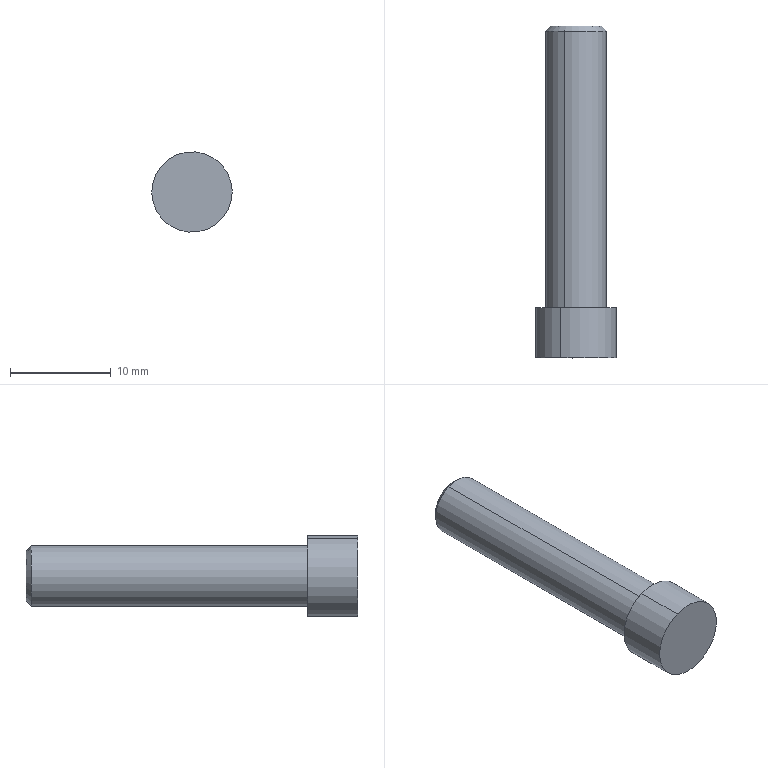Component | SolidWorks | 6x30TPunch-2 | 1 solid | 9 faces | box 8 x 33 x 8 mm | volume 1041 mm3 | cylinder 4 | plane 3 | cone 2 | commonest cylinder face diameters 8 x2 6 x2 | material Cr12
build123d program:
from build123d import *

# Parameters (mm, degrees)
SKETCH1_R           = 3
BOSS_EXTRUDE1_DEPTH = 28
SKETCH2_R           = 4
BOSS_EXTRUDE2_DEPTH = 5
CHAMFER1_SIZE       = 0.5


with BuildPart() as part:
    # Sketch1 → Boss-Extrude1 (new body)
    with BuildSketch(Plane(origin=(0, 0, 0), x_dir=(1, 0, 0), z_dir=(0, 1, 0))):
        with Locations(Location((0, 0, 0), (0, 0, 270))):
            Circle(SKETCH1_R)
    extrude(amount=BOSS_EXTRUDE1_DEPTH)

    # Sketch2 → Boss-Extrude2 (add)
    with BuildSketch(Plane(origin=(0, 28, 0), x_dir=(1, 0, 0), z_dir=(0, 1, 0))):
        with Locations(Location((0, 0, 0), (0, 0, 270))):
            Circle(SKETCH2_R)
    extrude(amount=BOSS_EXTRUDE2_DEPTH)

    # Chamfer1
    chamfer1_edges = [part.edges().sort_by_distance(p)[0] for p in [
        (0, 0, -3),
    ]]
    chamfer(chamfer1_edges, length=CHAMFER1_SIZE)


solid = part.part

# Placed as in the assembly
solid = solid.moved(Location((121.714, -49, 0), (180, 0, 0)))
STEP:
#1=CARTESIAN_POINT('',(4.829,-1.929,-0.09107));
#2=VERTEX_POINT('',#1);
#3=CARTESIAN_POINT('',(4.755,-1.929,0.09107));
#4=VERTEX_POINT('',#3);
#5=CARTESIAN_POINT('',(4.792,-1.929,-0.));
#6=DIRECTION('',(-0.,1.,0.));
#7=DIRECTION('',(-0.3794,0.,0.9252));
#8=AXIS2_PLACEMENT_3D('',#5,#6,#7);
#9=CIRCLE('',#8,0.09843);
#10=EDGE_CURVE('',#2,#4,#9,.T.);
#11=ORIENTED_EDGE('',*,*,#10,.F.);
#12=CARTESIAN_POINT('',(4.837,-1.949,-0.1093));
#13=VERTEX_POINT('',#12);
#14=CARTESIAN_POINT('',(4.837,-1.949,-0.1093));
#15=DIRECTION('',(0.2683,-0.7071,-0.6542));
#16=VECTOR('',#15,39.37);
#17=LINE('',#14,#16);
#18=EDGE_CURVE('',#2,#13,#17,.T.);
#19=ORIENTED_EDGE('',*,*,#18,.T.);
#20=CARTESIAN_POINT('',(4.747,-1.949,0.1093));
#21=VERTEX_POINT('',#20);
#22=CARTESIAN_POINT('',(4.792,-1.949,-0.));
#23=DIRECTION('',(0.,-1.,-0.));
#24=DIRECTION('',(-0.3794,0.,0.9252));
#25=AXIS2_PLACEMENT_3D('',#22,#23,#24);
#26=CIRCLE('',#25,0.1181);
#27=EDGE_CURVE('',#21,#13,#26,.T.);
#28=ORIENTED_EDGE('',*,*,#27,.F.);
#29=CARTESIAN_POINT('',(4.747,-1.949,0.1093));
#30=DIRECTION('',(-0.2683,-0.7071,0.6542));
#31=VECTOR('',#30,39.37);
#32=LINE('',#29,#31);
#33=EDGE_CURVE('',#4,#21,#32,.T.);
#34=ORIENTED_EDGE('',*,*,#33,.F.);
#35=EDGE_LOOP('',(#11,#19,#28,#34));
#36=FACE_OUTER_BOUND('',#35,.T.);
#37=CARTESIAN_POINT('',(4.792,-1.949,-0.));
#38=DIRECTION('',(0.,-1.,-0.));
#39=DIRECTION('',(-0.3794,0.,0.9252));
#40=AXIS2_PLACEMENT_3D('',#37,#38,#39);
#41=CONICAL_SURFACE('',#40,0.1181,0.7854);
#42=ADVANCED_FACE('',(#36),#41,.T.);
#43=CARTESIAN_POINT('',(4.732,-3.228,0.1457));
#44=VERTEX_POINT('',#43);
#45=CARTESIAN_POINT('',(4.852,-3.228,-0.1457));
#46=VERTEX_POINT('',#45);
#47=CARTESIAN_POINT('',(4.792,-3.228,-0.));
#48=DIRECTION('',(0.,-1.,-0.));
#49=DIRECTION('',(-0.3794,0.,0.9252));
#50=AXIS2_PLACEMENT_3D('',#47,#48,#49);
#51=CIRCLE('',#50,0.1575);
#52=EDGE_CURVE('',#44,#46,#51,.T.);
#53=ORIENTED_EDGE('',*,*,#52,.F.);
#54=CARTESIAN_POINT('',(4.732,-3.031,0.1457));
#55=VERTEX_POINT('',#54);
#56=CARTESIAN_POINT('',(4.732,-3.228,0.1457));
#57=DIRECTION('',(-0.,1.,0.));
#58=VECTOR('',#57,39.37);
#59=LINE('',#56,#58);
#60=EDGE_CURVE('',#44,#55,#59,.T.);
#61=ORIENTED_EDGE('',*,*,#60,.T.);
#62=CARTESIAN_POINT('',(4.852,-3.031,-0.1457));
#63=VERTEX_POINT('',#62);
#64=CARTESIAN_POINT('',(4.792,-3.031,-0.));
#65=DIRECTION('',(0.,-1.,-0.));
#66=DIRECTION('',(-0.3794,0.,0.9252));
#67=AXIS2_PLACEMENT_3D('',#64,#65,#66);
#68=CIRCLE('',#67,0.1575);
#69=EDGE_CURVE('',#55,#63,#68,.T.);
#70=ORIENTED_EDGE('',*,*,#69,.T.);
#71=CARTESIAN_POINT('',(4.852,-3.228,-0.1457));
#72=DIRECTION('',(-0.,1.,0.));
#73=VECTOR('',#72,39.37);
#74=LINE('',#71,#73);
#75=EDGE_CURVE('',#46,#63,#74,.T.);
#76=ORIENTED_EDGE('',*,*,#75,.F.);
#77=EDGE_LOOP('',(#53,#61,#70,#76));
#78=FACE_OUTER_BOUND('',#77,.T.);
#79=CARTESIAN_POINT('',(4.792,-3.228,-0.));
#80=DIRECTION('',(-0.,1.,0.));
#81=DIRECTION('',(0.3794,0.,-0.9252));
#82=AXIS2_PLACEMENT_3D('',#79,#80,#81);
#83=CYLINDRICAL_SURFACE('',#82,0.1575);
#84=ADVANCED_FACE('',(#78),#83,.T.);
#85=CARTESIAN_POINT('',(4.747,-3.031,0.1093));
#86=VERTEX_POINT('',#85);
#87=CARTESIAN_POINT('',(4.837,-3.031,-0.1093));
#88=VERTEX_POINT('',#87);
#89=CARTESIAN_POINT('',(4.792,-3.031,-0.));
#90=DIRECTION('',(0.,-1.,-0.));
#91=DIRECTION('',(-0.3794,0.,0.9252));
#92=AXIS2_PLACEMENT_3D('',#89,#90,#91);
#93=CIRCLE('',#92,0.1181);
#94=EDGE_CURVE('',#86,#88,#93,.T.);
#95=ORIENTED_EDGE('',*,*,#94,.F.);
#96=CARTESIAN_POINT('',(4.747,-3.031,0.1093));
#97=DIRECTION('',(-0.,1.,0.));
#98=VECTOR('',#97,39.37);
#99=LINE('',#96,#98);
#100=EDGE_CURVE('',#86,#21,#99,.T.);
#101=ORIENTED_EDGE('',*,*,#100,.T.);
#102=ORIENTED_EDGE('',*,*,#27,.T.);
#103=CARTESIAN_POINT('',(4.837,-3.031,-0.1093));
#104=DIRECTION('',(-0.,1.,0.));
#105=VECTOR('',#104,39.37);
#106=LINE('',#103,#105);
#107=EDGE_CURVE('',#88,#13,#106,.T.);
#108=ORIENTED_EDGE('',*,*,#107,.F.);
#109=EDGE_LOOP('',(#95,#101,#102,#108));
#110=FACE_OUTER_BOUND('',#109,.T.);
#111=CARTESIAN_POINT('',(4.792,-3.031,-0.));
#112=DIRECTION('',(-0.,1.,0.));
#113=DIRECTION('',(0.3794,0.,-0.9252));
#114=AXIS2_PLACEMENT_3D('',#111,#112,#113);
#115=CYLINDRICAL_SURFACE('',#114,0.1181);
#116=ADVANCED_FACE('',(#110),#115,.T.);
#117=ORIENTED_EDGE('',*,*,#100,.F.);
#118=CARTESIAN_POINT('',(4.792,-3.031,-0.));
#119=DIRECTION('',(0.,-1.,-0.));
#120=DIRECTION('',(-0.3794,0.,0.9252));
#121=AXIS2_PLACEMENT_3D('',#118,#119,#120);
#122=CIRCLE('',#121,0.1181);
#123=EDGE_CURVE('',#88,#86,#122,.T.);
#124=ORIENTED_EDGE('',*,*,#123,.F.);
#125=ORIENTED_EDGE('',*,*,#107,.T.);
#126=CARTESIAN_POINT('',(4.792,-1.949,-0.));
#127=DIRECTION('',(0.,-1.,-0.));
#128=DIRECTION('',(-0.3794,0.,0.9252));
#129=AXIS2_PLACEMENT_3D('',#126,#127,#128);
#130=CIRCLE('',#129,0.1181);
#131=EDGE_CURVE('',#13,#21,#130,.T.);
#132=ORIENTED_EDGE('',*,*,#131,.T.);
#133=EDGE_LOOP('',(#117,#124,#125,#132));
#134=FACE_OUTER_BOUND('',#133,.T.);
#135=CARTESIAN_POINT('',(4.792,-3.031,-0.));
#136=DIRECTION('',(-0.,1.,0.));
#137=DIRECTION('',(0.3794,0.,-0.9252));
#138=AXIS2_PLACEMENT_3D('',#135,#136,#137);
#139=CYLINDRICAL_SURFACE('',#138,0.1181);
#140=ADVANCED_FACE('',(#134),#139,.T.);
#141=CARTESIAN_POINT('',(4.792,-1.929,-0.));
#142=DIRECTION('',(-0.,1.,0.));
#143=DIRECTION('',(-0.3794,0.,0.9252));
#144=AXIS2_PLACEMENT_3D('',#141,#142,#143);
#145=CIRCLE('',#144,0.09843);
#146=EDGE_CURVE('',#4,#2,#145,.T.);
#147=ORIENTED_EDGE('',*,*,#146,.T.);
#148=ORIENTED_EDGE('',*,*,#10,.T.);
#149=EDGE_LOOP('',(#147,#148));
#150=FACE_OUTER_BOUND('',#149,.T.);
#151=CARTESIAN_POINT('',(4.792,-1.929,-0.));
#152=DIRECTION('',(-0.,-1.,-0.));
#153=DIRECTION('',(-0.3794,-0.,0.9252));
#154=AXIS2_PLACEMENT_3D('',#151,#152,#153);
#155=PLANE('',#154);
#156=ADVANCED_FACE('',(#150),#155,.F.);
#157=ORIENTED_EDGE('',*,*,#60,.F.);
#158=CARTESIAN_POINT('',(4.792,-3.228,-0.));
#159=DIRECTION('',(0.,-1.,-0.));
#160=DIRECTION('',(-0.3794,0.,0.9252));
#161=AXIS2_PLACEMENT_3D('',#158,#159,#160);
#162=CIRCLE('',#161,0.1575);
#163=EDGE_CURVE('',#46,#44,#162,.T.);
#164=ORIENTED_EDGE('',*,*,#163,.F.);
#165=ORIENTED_EDGE('',*,*,#75,.T.);
#166=CARTESIAN_POINT('',(4.792,-3.031,-0.));
#167=DIRECTION('',(0.,-1.,-0.));
#168=DIRECTION('',(-0.3794,0.,0.9252));
#169=AXIS2_PLACEMENT_3D('',#166,#167,#168);
#170=CIRCLE('',#169,0.1575);
#171=EDGE_CURVE('',#63,#55,#170,.T.);
#172=ORIENTED_EDGE('',*,*,#171,.T.);
#173=EDGE_LOOP('',(#157,#164,#165,#172));
#174=FACE_OUTER_BOUND('',#173,.T.);
#175=CARTESIAN_POINT('',(4.792,-3.228,-0.));
#176=DIRECTION('',(-0.,1.,0.));
#177=DIRECTION('',(0.3794,0.,-0.9252));
#178=AXIS2_PLACEMENT_3D('',#175,#176,#177);
#179=CYLINDRICAL_SURFACE('',#178,0.1575);
#180=ADVANCED_FACE('',(#174),#179,.T.);
#181=ORIENTED_EDGE('',*,*,#163,.T.);
#182=ORIENTED_EDGE('',*,*,#52,.T.);
#183=EDGE_LOOP('',(#181,#182));
#184=FACE_OUTER_BOUND('',#183,.T.);
#185=CARTESIAN_POINT('',(4.792,-3.228,-0.));
#186=DIRECTION('',(-0.,-1.,-0.));
#187=DIRECTION('',(-0.3794,-0.,0.9252));
#188=AXIS2_PLACEMENT_3D('',#185,#186,#187);
#189=PLANE('',#188);
#190=ADVANCED_FACE('',(#184),#189,.T.);
#191=ORIENTED_EDGE('',*,*,#123,.T.);
#192=ORIENTED_EDGE('',*,*,#94,.T.);
#193=EDGE_LOOP('',(#191,#192));
#194=FACE_BOUND('',#193,.T.);
#195=ORIENTED_EDGE('',*,*,#171,.F.);
#196=ORIENTED_EDGE('',*,*,#69,.F.);
#197=EDGE_LOOP('',(#195,#196));
#198=FACE_OUTER_BOUND('',#197,.T.);
#199=CARTESIAN_POINT('',(4.792,-3.031,-0.));
#200=DIRECTION('',(-0.,-1.,-0.));
#201=DIRECTION('',(-0.3794,-0.,0.9252));
#202=AXIS2_PLACEMENT_3D('',#199,#200,#201);
#203=PLANE('',#202);
#204=ADVANCED_FACE('',(#194,#198),#203,.F.);
#205=ORIENTED_EDGE('',*,*,#18,.F.);
#206=ORIENTED_EDGE('',*,*,#146,.F.);
#207=ORIENTED_EDGE('',*,*,#33,.T.);
#208=ORIENTED_EDGE('',*,*,#131,.F.);
#209=EDGE_LOOP('',(#205,#206,#207,#208));
#210=FACE_OUTER_BOUND('',#209,.T.);
#211=CARTESIAN_POINT('',(4.792,-1.949,-0.));
#212=DIRECTION('',(0.,-1.,-0.));
#213=DIRECTION('',(-0.3794,0.,0.9252));
#214=AXIS2_PLACEMENT_3D('',#211,#212,#213);
#215=CONICAL_SURFACE('',#214,0.1181,0.7854);
#216=ADVANCED_FACE('',(#210),#215,.T.);
#217=CLOSED_SHELL('',(#42,#84,#116,#140,#156,#180,#190,#204,#216));
#218=MANIFOLD_SOLID_BREP('',#217);
#219=CARTESIAN_POINT('',(0.,0.,0.));
#220=DIRECTION('',(0.,0.,1.));
#221=DIRECTION('',(1.,0.,0.));
#222=AXIS2_PLACEMENT_3D('',#219,#220,#221);
#223=(LENGTH_UNIT()NAMED_UNIT(*)SI_UNIT($,.METRE.));
#224=LENGTH_MEASURE_WITH_UNIT(LENGTH_MEASURE(0.0254),#223);
#225=DIMENSIONAL_EXPONENTS(1.,0.,0.,0.,0.,0.,0.);
#226=(CONVERSION_BASED_UNIT('',#224)LENGTH_UNIT()NAMED_UNIT(#225));
#227=UNCERTAINTY_MEASURE_WITH_UNIT(LENGTH_MEASURE(0.00001),#226,'','');
#228=(NAMED_UNIT(*)PLANE_ANGLE_UNIT()SI_UNIT($,.RADIAN.));
#229=(NAMED_UNIT(*)SI_UNIT($,.STERADIAN.)SOLID_ANGLE_UNIT());
#230=(GEOMETRIC_REPRESENTATION_CONTEXT(3)GLOBAL_UNCERTAINTY_ASSIGNED_CONTEXT((#227))GLOBAL_UNIT_ASSIGNED_CONTEXT((#226,#228,#229))REPRESENTATION_CONTEXT('',''));
#231=ADVANCED_BREP_SHAPE_REPRESENTATION('',(#218,#222),#230);
#232=COLOUR_RGB('',0.7922,0.8196,0.9333);
#233=FILL_AREA_STYLE_COLOUR('',#232);
#234=FILL_AREA_STYLE('',(#233));
#235=SURFACE_STYLE_FILL_AREA(#234);
#236=SURFACE_SIDE_STYLE('',(#235));
#237=SURFACE_STYLE_USAGE(.BOTH.,#236);
#238=PRESENTATION_STYLE_ASSIGNMENT((#237));
#239=STYLED_ITEM('',(#238),#218);
#240=PRESENTATION_LAYER_ASSIGNMENT('','',(#239));
#241=(LENGTH_UNIT()NAMED_UNIT(*)SI_UNIT($,.METRE.));
#242=LENGTH_MEASURE_WITH_UNIT(LENGTH_MEASURE(0.0254),#241);
#243=DIMENSIONAL_EXPONENTS(1.,0.,0.,0.,0.,0.,0.);
#244=(CONVERSION_BASED_UNIT('',#242)LENGTH_UNIT()NAMED_UNIT(#243));
#245=UNCERTAINTY_MEASURE_WITH_UNIT(LENGTH_MEASURE(0.00001),#244,'','');
#246=(NAMED_UNIT(*)PLANE_ANGLE_UNIT()SI_UNIT($,.RADIAN.));
#247=(NAMED_UNIT(*)SI_UNIT($,.STERADIAN.)SOLID_ANGLE_UNIT());
#248=(GEOMETRIC_REPRESENTATION_CONTEXT(3)GLOBAL_UNCERTAINTY_ASSIGNED_CONTEXT((#245))GLOBAL_UNIT_ASSIGNED_CONTEXT((#244,#246,#247))REPRESENTATION_CONTEXT('',''));
#249=MECHANICAL_DESIGN_GEOMETRIC_PRESENTATION_REPRESENTATION('',(#239),#248);